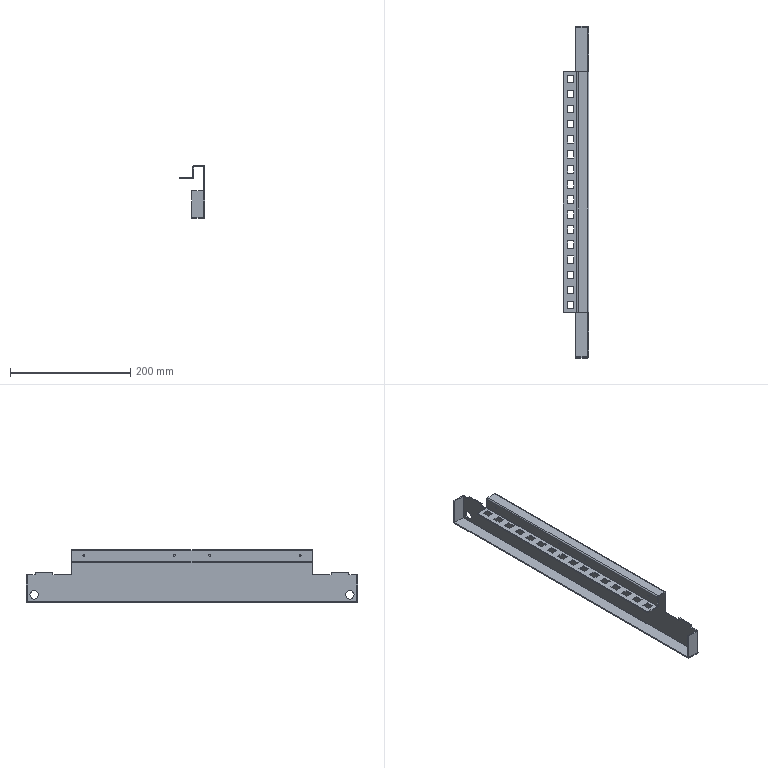Component | SolidWorks | CabinetFrameWeldmentDrawingPG50-01-00-1_BaseWeldingDrawingPG50-05-1_BaseWeldment1(PG50-05-101-2 | 1 solid | 144 faces | volume 151592 mm3 | plane 120 | cylinder 24 | commonest cylinder face diameters 3.2 x8 0.2 x6 4.2 x6 14 x4 | material AISI 1045 Steel, cold drawn